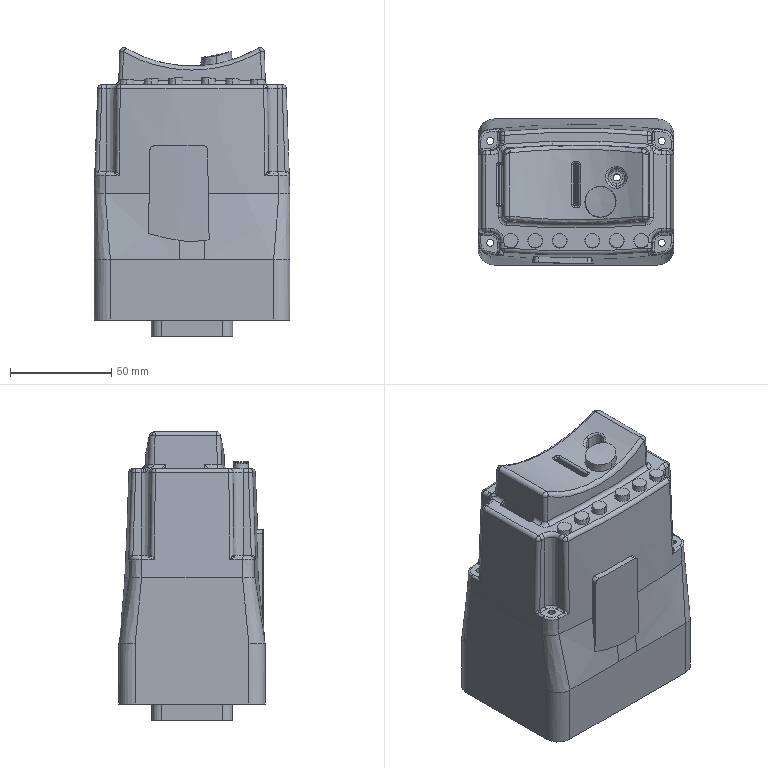CAM job | NX | mm | 3-axis | 1 set-up | 3 operations | part box 96.53 x 72 x 142.21
set-up 1
1. Cavity Milling | Mill Mill5 D12 | CAVITY_MILL | path 227495.445 mm | 77.585 min
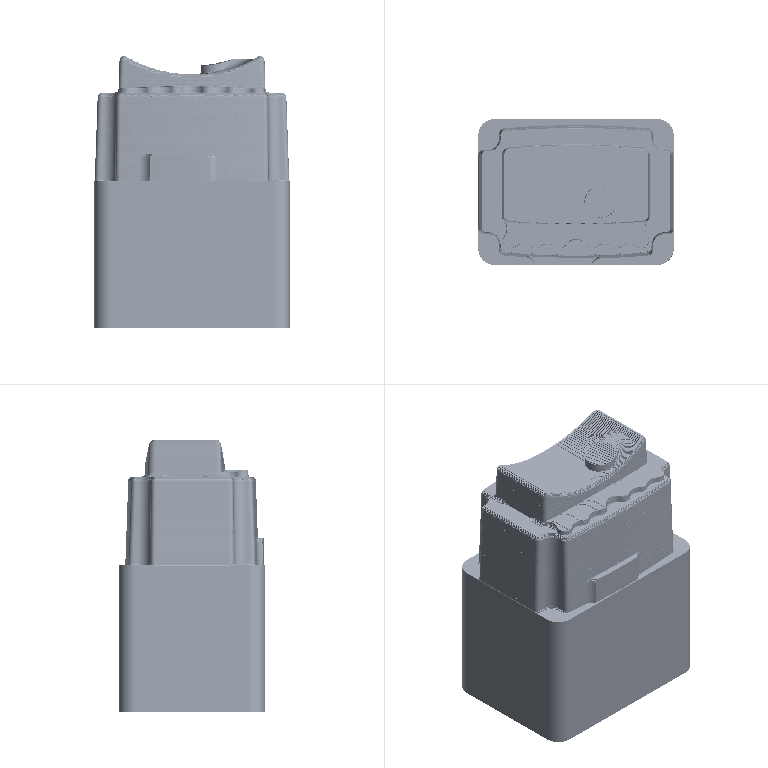2. Z-Level Milling | Mill Mill5 D12 | ZLEVEL_PROFILE | path 17795.745 mm | 7.074 min
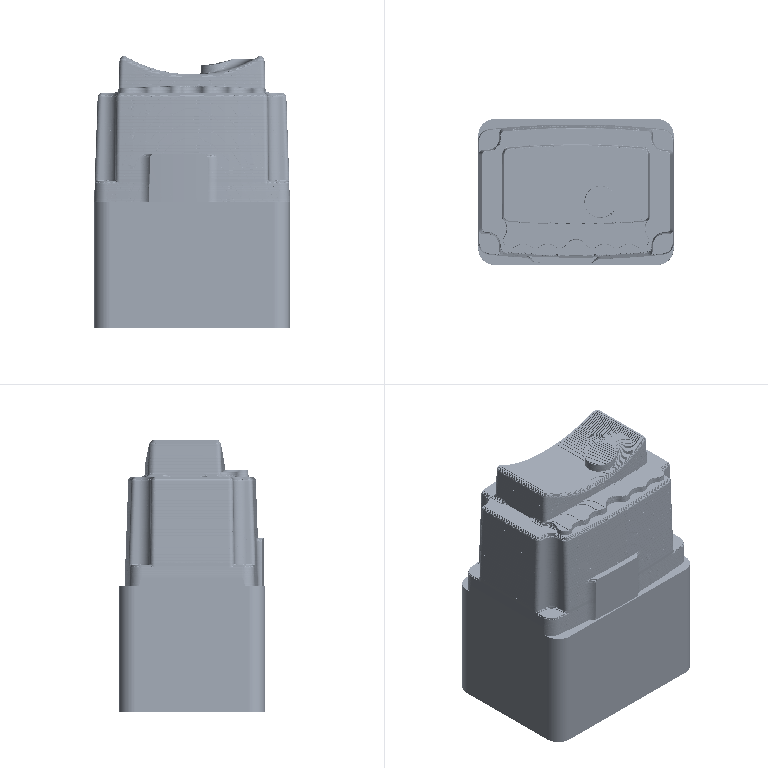3. Cavity Milling | Mill Mill5 D4 | CAVITY_MILL_1 | path 20380.588 mm | 8.135 min